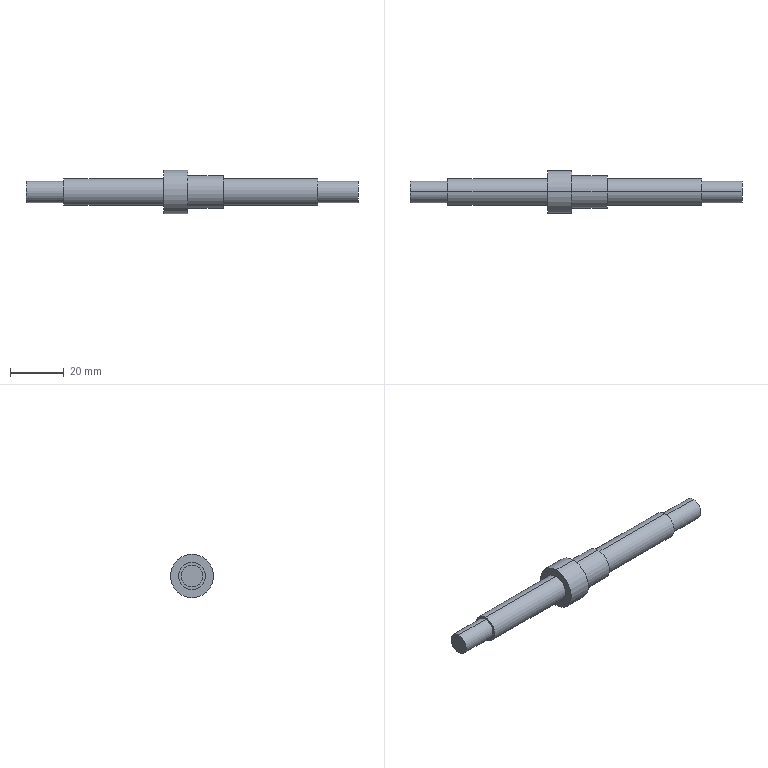Component | SolidWorks | IntermediateAxis-1 | 1 solid | 19 faces | box 123 x 16 x 16 mm | volume 10392 mm3 | cylinder 12 | plane 7 | commonest cylinder face diameters 8 x4 10 x4 12 x2 16 x2 | material AISI 1045 Steel, Cold Drawn
build123d program:
from build123d import *


with BuildPart() as part:
    # Sketch1 → Revolve1 (revolve)
    with BuildSketch(Plane.XY, mode=Mode.PRIVATE) as revolve1_sk:
        Polygon((0, 0), (0, 4), (14, 4), (14, 5), (51, 5), (51, 8), (60, 8), (60, 6), (73, 6), (73, 5), (108, 5), (108, 4), (123, 4), (123, 0), align=None)
    revolve(revolve1_sk.sketch.rotate(Axis((-147.307, 0, 0), (1, 0, 0)), 90), axis=Axis((-147.307, 0, 0), (1, 0, 0)))


solid = part.part

# Placed as in the assembly
solid = solid.moved(Location((116.062, 15.116, 349), (0, 0, 0)))
STEP:
#1=COLOUR_RGB('',0.7922,0.8196,0.9333);
#2=FILL_AREA_STYLE_COLOUR('',#1);
#3=FILL_AREA_STYLE('',(#2));
#4=SURFACE_STYLE_FILL_AREA(#3);
#5=SURFACE_SIDE_STYLE('',(#4));
#6=SURFACE_STYLE_USAGE(.BOTH.,#5);
#7=PRESENTATION_STYLE_ASSIGNMENT((#6));
#8=CARTESIAN_POINT('',(9.412,0.5951,13.898));
#9=VERTEX_POINT('',#8);
#10=CARTESIAN_POINT('',(9.412,0.5951,13.583));
#11=VERTEX_POINT('',#10);
#12=CARTESIAN_POINT('',(9.412,0.5951,13.74));
#13=DIRECTION('',(-1.,0.,0.));
#14=DIRECTION('',(0.,0.,1.));
#15=AXIS2_PLACEMENT_3D('',#12,#13,#14);
#16=CIRCLE('',#15,0.1575);
#17=EDGE_CURVE('',#9,#11,#16,.T.);
#18=ORIENTED_EDGE('',*,*,#17,.T.);
#19=CARTESIAN_POINT('',(8.821,0.5951,13.583));
#20=VERTEX_POINT('',#19);
#21=CARTESIAN_POINT('',(-1.23,0.5951,13.583));
#22=DIRECTION('',(-1.,0.,0.));
#23=VECTOR('',#22,39.37);
#24=LINE('',#21,#23);
#25=EDGE_CURVE('',#11,#20,#24,.T.);
#26=ORIENTED_EDGE('',*,*,#25,.T.);
#27=CARTESIAN_POINT('',(8.821,0.5951,13.898));
#28=VERTEX_POINT('',#27);
#29=CARTESIAN_POINT('',(8.821,0.5951,13.74));
#30=DIRECTION('',(-1.,0.,0.));
#31=DIRECTION('',(0.,0.,1.));
#32=AXIS2_PLACEMENT_3D('',#29,#30,#31);
#33=CIRCLE('',#32,0.1575);
#34=EDGE_CURVE('',#28,#20,#33,.T.);
#35=ORIENTED_EDGE('',*,*,#34,.F.);
#36=CARTESIAN_POINT('',(-1.23,0.5951,13.898));
#37=DIRECTION('',(-1.,0.,0.));
#38=VECTOR('',#37,39.37);
#39=LINE('',#36,#38);
#40=EDGE_CURVE('',#9,#28,#39,.T.);
#41=ORIENTED_EDGE('',*,*,#40,.F.);
#42=EDGE_LOOP('',(#18,#26,#35,#41));
#43=FACE_OUTER_BOUND('',#42,.T.);
#44=CARTESIAN_POINT('',(-1.23,0.5951,13.74));
#45=DIRECTION('',(-1.,0.,0.));
#46=DIRECTION('',(0.,0.,1.));
#47=AXIS2_PLACEMENT_3D('',#44,#45,#46);
#48=CYLINDRICAL_SURFACE('',#47,0.1575);
#49=ADVANCED_FACE('',(#43),#48,.T.);
#50=CARTESIAN_POINT('',(8.821,0.5951,13.937));
#51=VERTEX_POINT('',#50);
#52=CARTESIAN_POINT('',(8.821,0.5951,13.543));
#53=VERTEX_POINT('',#52);
#54=CARTESIAN_POINT('',(8.821,0.5951,13.74));
#55=DIRECTION('',(-1.,0.,0.));
#56=DIRECTION('',(0.,0.,1.));
#57=AXIS2_PLACEMENT_3D('',#54,#55,#56);
#58=CIRCLE('',#57,0.1969);
#59=EDGE_CURVE('',#51,#53,#58,.T.);
#60=ORIENTED_EDGE('',*,*,#59,.T.);
#61=CARTESIAN_POINT('',(7.443,0.5951,13.543));
#62=VERTEX_POINT('',#61);
#63=CARTESIAN_POINT('',(-1.23,0.5951,13.543));
#64=DIRECTION('',(-1.,0.,0.));
#65=VECTOR('',#64,39.37);
#66=LINE('',#63,#65);
#67=EDGE_CURVE('',#53,#62,#66,.T.);
#68=ORIENTED_EDGE('',*,*,#67,.T.);
#69=CARTESIAN_POINT('',(7.443,0.5951,13.937));
#70=VERTEX_POINT('',#69);
#71=CARTESIAN_POINT('',(7.443,0.5951,13.74));
#72=DIRECTION('',(-1.,0.,0.));
#73=DIRECTION('',(0.,0.,1.));
#74=AXIS2_PLACEMENT_3D('',#71,#72,#73);
#75=CIRCLE('',#74,0.1969);
#76=EDGE_CURVE('',#70,#62,#75,.T.);
#77=ORIENTED_EDGE('',*,*,#76,.F.);
#78=CARTESIAN_POINT('',(-1.23,0.5951,13.937));
#79=DIRECTION('',(-1.,0.,0.));
#80=VECTOR('',#79,39.37);
#81=LINE('',#78,#80);
#82=EDGE_CURVE('',#51,#70,#81,.T.);
#83=ORIENTED_EDGE('',*,*,#82,.F.);
#84=EDGE_LOOP('',(#60,#68,#77,#83));
#85=FACE_OUTER_BOUND('',#84,.T.);
#86=CARTESIAN_POINT('',(-1.23,0.5951,13.74));
#87=DIRECTION('',(-1.,0.,0.));
#88=DIRECTION('',(0.,0.,1.));
#89=AXIS2_PLACEMENT_3D('',#86,#87,#88);
#90=CYLINDRICAL_SURFACE('',#89,0.1969);
#91=ADVANCED_FACE('',(#85),#90,.T.);
#92=CARTESIAN_POINT('',(7.443,0.5951,13.976));
#93=VERTEX_POINT('',#92);
#94=CARTESIAN_POINT('',(7.443,0.5951,13.504));
#95=VERTEX_POINT('',#94);
#96=CARTESIAN_POINT('',(7.443,0.5951,13.74));
#97=DIRECTION('',(-1.,0.,0.));
#98=DIRECTION('',(0.,0.,1.));
#99=AXIS2_PLACEMENT_3D('',#96,#97,#98);
#100=CIRCLE('',#99,0.2362);
#101=EDGE_CURVE('',#93,#95,#100,.T.);
#102=ORIENTED_EDGE('',*,*,#101,.T.);
#103=CARTESIAN_POINT('',(6.932,0.5951,13.504));
#104=VERTEX_POINT('',#103);
#105=CARTESIAN_POINT('',(-1.23,0.5951,13.504));
#106=DIRECTION('',(-1.,0.,0.));
#107=VECTOR('',#106,39.37);
#108=LINE('',#105,#107);
#109=EDGE_CURVE('',#95,#104,#108,.T.);
#110=ORIENTED_EDGE('',*,*,#109,.T.);
#111=CARTESIAN_POINT('',(6.932,0.5951,13.976));
#112=VERTEX_POINT('',#111);
#113=CARTESIAN_POINT('',(6.932,0.5951,13.74));
#114=DIRECTION('',(-1.,0.,0.));
#115=DIRECTION('',(0.,0.,1.));
#116=AXIS2_PLACEMENT_3D('',#113,#114,#115);
#117=CIRCLE('',#116,0.2362);
#118=EDGE_CURVE('',#112,#104,#117,.T.);
#119=ORIENTED_EDGE('',*,*,#118,.F.);
#120=CARTESIAN_POINT('',(-1.23,0.5951,13.976));
#121=DIRECTION('',(-1.,0.,0.));
#122=VECTOR('',#121,39.37);
#123=LINE('',#120,#122);
#124=EDGE_CURVE('',#93,#112,#123,.T.);
#125=ORIENTED_EDGE('',*,*,#124,.F.);
#126=EDGE_LOOP('',(#102,#110,#119,#125));
#127=FACE_OUTER_BOUND('',#126,.T.);
#128=CARTESIAN_POINT('',(-1.23,0.5951,13.74));
#129=DIRECTION('',(-1.,0.,0.));
#130=DIRECTION('',(0.,0.,1.));
#131=AXIS2_PLACEMENT_3D('',#128,#129,#130);
#132=CYLINDRICAL_SURFACE('',#131,0.2362);
#133=ADVANCED_FACE('',(#127),#132,.T.);
#134=CARTESIAN_POINT('',(6.932,0.5951,14.055));
#135=VERTEX_POINT('',#134);
#136=CARTESIAN_POINT('',(6.932,0.5951,13.425));
#137=VERTEX_POINT('',#136);
#138=CARTESIAN_POINT('',(6.932,0.5951,13.74));
#139=DIRECTION('',(-1.,0.,0.));
#140=DIRECTION('',(0.,0.,1.));
#141=AXIS2_PLACEMENT_3D('',#138,#139,#140);
#142=CIRCLE('',#141,0.315);
#143=EDGE_CURVE('',#135,#137,#142,.T.);
#144=ORIENTED_EDGE('',*,*,#143,.T.);
#145=CARTESIAN_POINT('',(6.577,0.5951,13.425));
#146=VERTEX_POINT('',#145);
#147=CARTESIAN_POINT('',(-1.23,0.5951,13.425));
#148=DIRECTION('',(-1.,0.,0.));
#149=VECTOR('',#148,39.37);
#150=LINE('',#147,#149);
#151=EDGE_CURVE('',#137,#146,#150,.T.);
#152=ORIENTED_EDGE('',*,*,#151,.T.);
#153=CARTESIAN_POINT('',(6.577,0.5951,14.055));
#154=VERTEX_POINT('',#153);
#155=CARTESIAN_POINT('',(6.577,0.5951,13.74));
#156=DIRECTION('',(-1.,0.,0.));
#157=DIRECTION('',(0.,0.,1.));
#158=AXIS2_PLACEMENT_3D('',#155,#156,#157);
#159=CIRCLE('',#158,0.315);
#160=EDGE_CURVE('',#154,#146,#159,.T.);
#161=ORIENTED_EDGE('',*,*,#160,.F.);
#162=CARTESIAN_POINT('',(-1.23,0.5951,14.055));
#163=DIRECTION('',(-1.,0.,0.));
#164=VECTOR('',#163,39.37);
#165=LINE('',#162,#164);
#166=EDGE_CURVE('',#135,#154,#165,.T.);
#167=ORIENTED_EDGE('',*,*,#166,.F.);
#168=EDGE_LOOP('',(#144,#152,#161,#167));
#169=FACE_OUTER_BOUND('',#168,.T.);
#170=CARTESIAN_POINT('',(-1.23,0.5951,13.74));
#171=DIRECTION('',(-1.,0.,0.));
#172=DIRECTION('',(0.,0.,1.));
#173=AXIS2_PLACEMENT_3D('',#170,#171,#172);
#174=CYLINDRICAL_SURFACE('',#173,0.315);
#175=ADVANCED_FACE('',(#169),#174,.T.);
#176=CARTESIAN_POINT('',(6.577,0.5951,13.937));
#177=VERTEX_POINT('',#176);
#178=CARTESIAN_POINT('',(6.577,0.5951,13.543));
#179=VERTEX_POINT('',#178);
#180=CARTESIAN_POINT('',(6.577,0.5951,13.74));
#181=DIRECTION('',(-1.,0.,0.));
#182=DIRECTION('',(0.,0.,1.));
#183=AXIS2_PLACEMENT_3D('',#180,#181,#182);
#184=CIRCLE('',#183,0.1969);
#185=EDGE_CURVE('',#177,#179,#184,.T.);
#186=ORIENTED_EDGE('',*,*,#185,.T.);
#187=CARTESIAN_POINT('',(5.121,0.5951,13.543));
#188=VERTEX_POINT('',#187);
#189=CARTESIAN_POINT('',(-1.23,0.5951,13.543));
#190=DIRECTION('',(-1.,0.,0.));
#191=VECTOR('',#190,39.37);
#192=LINE('',#189,#191);
#193=EDGE_CURVE('',#179,#188,#192,.T.);
#194=ORIENTED_EDGE('',*,*,#193,.T.);
#195=CARTESIAN_POINT('',(5.121,0.5951,13.937));
#196=VERTEX_POINT('',#195);
#197=CARTESIAN_POINT('',(5.121,0.5951,13.74));
#198=DIRECTION('',(-1.,0.,0.));
#199=DIRECTION('',(0.,0.,1.));
#200=AXIS2_PLACEMENT_3D('',#197,#198,#199);
#201=CIRCLE('',#200,0.1969);
#202=EDGE_CURVE('',#196,#188,#201,.T.);
#203=ORIENTED_EDGE('',*,*,#202,.F.);
#204=CARTESIAN_POINT('',(-1.23,0.5951,13.937));
#205=DIRECTION('',(-1.,0.,0.));
#206=VECTOR('',#205,39.37);
#207=LINE('',#204,#206);
#208=EDGE_CURVE('',#177,#196,#207,.T.);
#209=ORIENTED_EDGE('',*,*,#208,.F.);
#210=EDGE_LOOP('',(#186,#194,#203,#209));
#211=FACE_OUTER_BOUND('',#210,.T.);
#212=CARTESIAN_POINT('',(-1.23,0.5951,13.74));
#213=DIRECTION('',(-1.,0.,0.));
#214=DIRECTION('',(0.,0.,1.));
#215=AXIS2_PLACEMENT_3D('',#212,#213,#214);
#216=CYLINDRICAL_SURFACE('',#215,0.1969);
#217=ADVANCED_FACE('',(#211),#216,.T.);
#218=CARTESIAN_POINT('',(5.121,0.5951,13.898));
#219=VERTEX_POINT('',#218);
#220=CARTESIAN_POINT('',(5.121,0.5951,13.583));
#221=VERTEX_POINT('',#220);
#222=CARTESIAN_POINT('',(5.121,0.5951,13.74));
#223=DIRECTION('',(-1.,0.,0.));
#224=DIRECTION('',(0.,0.,1.));
#225=AXIS2_PLACEMENT_3D('',#222,#223,#224);
#226=CIRCLE('',#225,0.1575);
#227=EDGE_CURVE('',#219,#221,#226,.T.);
#228=ORIENTED_EDGE('',*,*,#227,.T.);
#229=CARTESIAN_POINT('',(4.569,0.5951,13.583));
#230=VERTEX_POINT('',#229);
#231=CARTESIAN_POINT('',(-1.23,0.5951,13.583));
#232=DIRECTION('',(-1.,0.,0.));
#233=VECTOR('',#232,39.37);
#234=LINE('',#231,#233);
#235=EDGE_CURVE('',#221,#230,#234,.T.);
#236=ORIENTED_EDGE('',*,*,#235,.T.);
#237=CARTESIAN_POINT('',(4.569,0.5951,13.898));
#238=VERTEX_POINT('',#237);
#239=CARTESIAN_POINT('',(4.569,0.5951,13.74));
#240=DIRECTION('',(-1.,0.,0.));
#241=DIRECTION('',(0.,0.,1.));
#242=AXIS2_PLACEMENT_3D('',#239,#240,#241);
#243=CIRCLE('',#242,0.1575);
#244=EDGE_CURVE('',#238,#230,#243,.T.);
#245=ORIENTED_EDGE('',*,*,#244,.F.);
#246=CARTESIAN_POINT('',(-1.23,0.5951,13.898));
#247=DIRECTION('',(-1.,0.,0.));
#248=VECTOR('',#247,39.37);
#249=LINE('',#246,#248);
#250=EDGE_CURVE('',#219,#238,#249,.T.);
#251=ORIENTED_EDGE('',*,*,#250,.F.);
#252=EDGE_LOOP('',(#228,#236,#245,#251));
#253=FACE_OUTER_BOUND('',#252,.T.);
#254=CARTESIAN_POINT('',(-1.23,0.5951,13.74));
#255=DIRECTION('',(-1.,0.,0.));
#256=DIRECTION('',(0.,0.,1.));
#257=AXIS2_PLACEMENT_3D('',#254,#255,#256);
#258=CYLINDRICAL_SURFACE('',#257,0.1575);
#259=ADVANCED_FACE('',(#253),#258,.T.);
#260=ORIENTED_EDGE('',*,*,#244,.T.);
#261=CARTESIAN_POINT('',(4.569,0.5951,13.74));
#262=DIRECTION('',(-1.,0.,0.));
#263=DIRECTION('',(0.,0.,1.));
#264=AXIS2_PLACEMENT_3D('',#261,#262,#263);
#265=CIRCLE('',#264,0.1575);
#266=EDGE_CURVE('',#230,#238,#265,.T.);
#267=ORIENTED_EDGE('',*,*,#266,.T.);
#268=EDGE_LOOP('',(#260,#267));
#269=FACE_OUTER_BOUND('',#268,.T.);
#270=CARTESIAN_POINT('',(4.569,0.5951,13.74));
#271=DIRECTION('',(1.,0.,0.));
#272=DIRECTION('',(0.,0.,-1.));
#273=AXIS2_PLACEMENT_3D('',#270,#271,#272);
#274=PLANE('',#273);
#275=ADVANCED_FACE('',(#269),#274,.F.);
#276=ORIENTED_EDGE('',*,*,#235,.F.);
#277=CARTESIAN_POINT('',(5.121,0.5951,13.74));
#278=DIRECTION('',(-1.,0.,0.));
#279=DIRECTION('',(0.,0.,1.));
#280=AXIS2_PLACEMENT_3D('',#277,#278,#279);
#281=CIRCLE('',#280,0.1575);
#282=EDGE_CURVE('',#221,#219,#281,.T.);
#283=ORIENTED_EDGE('',*,*,#282,.T.);
#284=ORIENTED_EDGE('',*,*,#250,.T.);
#285=ORIENTED_EDGE('',*,*,#266,.F.);
#286=EDGE_LOOP('',(#276,#283,#284,#285));
#287=FACE_OUTER_BOUND('',#286,.T.);
#288=CARTESIAN_POINT('',(-1.23,0.5951,13.74));
#289=DIRECTION('',(-1.,0.,0.));
#290=DIRECTION('',(0.,0.,1.));
#291=AXIS2_PLACEMENT_3D('',#288,#289,#290);
#292=CYLINDRICAL_SURFACE('',#291,0.1575);
#293=ADVANCED_FACE('',(#287),#292,.T.);
#294=ORIENTED_EDGE('',*,*,#227,.F.);
#295=ORIENTED_EDGE('',*,*,#282,.F.);
#296=EDGE_LOOP('',(#294,#295));
#297=FACE_BOUND('',#296,.T.);
#298=ORIENTED_EDGE('',*,*,#202,.T.);
#299=CARTESIAN_POINT('',(5.121,0.5951,13.74));
#300=DIRECTION('',(-1.,0.,0.));
#301=DIRECTION('',(0.,0.,1.));
#302=AXIS2_PLACEMENT_3D('',#299,#300,#301);
#303=CIRCLE('',#302,0.1969);
#304=EDGE_CURVE('',#188,#196,#303,.T.);
#305=ORIENTED_EDGE('',*,*,#304,.T.);
#306=EDGE_LOOP('',(#298,#305));
#307=FACE_OUTER_BOUND('',#306,.T.);
#308=CARTESIAN_POINT('',(5.121,0.7526,13.74));
#309=DIRECTION('',(1.,0.,0.));
#310=DIRECTION('',(0.,0.,-1.));
#311=AXIS2_PLACEMENT_3D('',#308,#309,#310);
#312=PLANE('',#311);
#313=ADVANCED_FACE('',(#297,#307),#312,.F.);
#314=ORIENTED_EDGE('',*,*,#193,.F.);
#315=CARTESIAN_POINT('',(6.577,0.5951,13.74));
#316=DIRECTION('',(-1.,0.,0.));
#317=DIRECTION('',(0.,0.,1.));
#318=AXIS2_PLACEMENT_3D('',#315,#316,#317);
#319=CIRCLE('',#318,0.1969);
#320=EDGE_CURVE('',#179,#177,#319,.T.);
#321=ORIENTED_EDGE('',*,*,#320,.T.);
#322=ORIENTED_EDGE('',*,*,#208,.T.);
#323=ORIENTED_EDGE('',*,*,#304,.F.);
#324=EDGE_LOOP('',(#314,#321,#322,#323));
#325=FACE_OUTER_BOUND('',#324,.T.);
#326=CARTESIAN_POINT('',(-1.23,0.5951,13.74));
#327=DIRECTION('',(-1.,0.,0.));
#328=DIRECTION('',(0.,0.,1.));
#329=AXIS2_PLACEMENT_3D('',#326,#327,#328);
#330=CYLINDRICAL_SURFACE('',#329,0.1969);
#331=ADVANCED_FACE('',(#325),#330,.T.);
#332=ORIENTED_EDGE('',*,*,#185,.F.);
#333=ORIENTED_EDGE('',*,*,#320,.F.);
#334=EDGE_LOOP('',(#332,#333));
#335=FACE_BOUND('',#334,.T.);
#336=ORIENTED_EDGE('',*,*,#160,.T.);
#337=CARTESIAN_POINT('',(6.577,0.5951,13.74));
#338=DIRECTION('',(-1.,0.,0.));
#339=DIRECTION('',(0.,0.,1.));
#340=AXIS2_PLACEMENT_3D('',#337,#338,#339);
#341=CIRCLE('',#340,0.315);
#342=EDGE_CURVE('',#146,#154,#341,.T.);
#343=ORIENTED_EDGE('',*,*,#342,.T.);
#344=EDGE_LOOP('',(#336,#343));
#345=FACE_OUTER_BOUND('',#344,.T.);
#346=CARTESIAN_POINT('',(6.577,0.792,13.74));
#347=DIRECTION('',(1.,0.,0.));
#348=DIRECTION('',(0.,0.,-1.));
#349=AXIS2_PLACEMENT_3D('',#346,#347,#348);
#350=PLANE('',#349);
#351=ADVANCED_FACE('',(#335,#345),#350,.F.);
#352=ORIENTED_EDGE('',*,*,#151,.F.);
#353=CARTESIAN_POINT('',(6.932,0.5951,13.74));
#354=DIRECTION('',(-1.,0.,0.));
#355=DIRECTION('',(0.,0.,1.));
#356=AXIS2_PLACEMENT_3D('',#353,#354,#355);
#357=CIRCLE('',#356,0.315);
#358=EDGE_CURVE('',#137,#135,#357,.T.);
#359=ORIENTED_EDGE('',*,*,#358,.T.);
#360=ORIENTED_EDGE('',*,*,#166,.T.);
#361=ORIENTED_EDGE('',*,*,#342,.F.);
#362=EDGE_LOOP('',(#352,#359,#360,#361));
#363=FACE_OUTER_BOUND('',#362,.T.);
#364=CARTESIAN_POINT('',(-1.23,0.5951,13.74));
#365=DIRECTION('',(-1.,0.,0.));
#366=DIRECTION('',(0.,0.,1.));
#367=AXIS2_PLACEMENT_3D('',#364,#365,#366);
#368=CYLINDRICAL_SURFACE('',#367,0.315);
#369=ADVANCED_FACE('',(#363),#368,.T.);
#370=ORIENTED_EDGE('',*,*,#143,.F.);
#371=ORIENTED_EDGE('',*,*,#358,.F.);
#372=EDGE_LOOP('',(#370,#371));
#373=FACE_OUTER_BOUND('',#372,.T.);
#374=ORIENTED_EDGE('',*,*,#118,.T.);
#375=CARTESIAN_POINT('',(6.932,0.5951,13.74));
#376=DIRECTION('',(-1.,0.,0.));
#377=DIRECTION('',(0.,0.,1.));
#378=AXIS2_PLACEMENT_3D('',#375,#376,#377);
#379=CIRCLE('',#378,0.2362);
#380=EDGE_CURVE('',#104,#112,#379,.T.);
#381=ORIENTED_EDGE('',*,*,#380,.T.);
#382=EDGE_LOOP('',(#374,#381));
#383=FACE_BOUND('',#382,.T.);
#384=CARTESIAN_POINT('',(6.932,0.9101,13.74));
#385=DIRECTION('',(-1.,0.,0.));
#386=DIRECTION('',(0.,0.,1.));
#387=AXIS2_PLACEMENT_3D('',#384,#385,#386);
#388=PLANE('',#387);
#389=ADVANCED_FACE('',(#373,#383),#388,.F.);
#390=ORIENTED_EDGE('',*,*,#109,.F.);
#391=CARTESIAN_POINT('',(7.443,0.5951,13.74));
#392=DIRECTION('',(-1.,0.,0.));
#393=DIRECTION('',(0.,0.,1.));
#394=AXIS2_PLACEMENT_3D('',#391,#392,#393);
#395=CIRCLE('',#394,0.2362);
#396=EDGE_CURVE('',#95,#93,#395,.T.);
#397=ORIENTED_EDGE('',*,*,#396,.T.);
#398=ORIENTED_EDGE('',*,*,#124,.T.);
#399=ORIENTED_EDGE('',*,*,#380,.F.);
#400=EDGE_LOOP('',(#390,#397,#398,#399));
#401=FACE_OUTER_BOUND('',#400,.T.);
#402=CARTESIAN_POINT('',(-1.23,0.5951,13.74));
#403=DIRECTION('',(-1.,0.,0.));
#404=DIRECTION('',(0.,0.,1.));
#405=AXIS2_PLACEMENT_3D('',#402,#403,#404);
#406=CYLINDRICAL_SURFACE('',#405,0.2362);
#407=ADVANCED_FACE('',(#401),#406,.T.);
#408=ORIENTED_EDGE('',*,*,#101,.F.);
#409=ORIENTED_EDGE('',*,*,#396,.F.);
#410=EDGE_LOOP('',(#408,#409));
#411=FACE_OUTER_BOUND('',#410,.T.);
#412=ORIENTED_EDGE('',*,*,#76,.T.);
#413=CARTESIAN_POINT('',(7.443,0.5951,13.74));
#414=DIRECTION('',(-1.,0.,0.));
#415=DIRECTION('',(0.,0.,1.));
#416=AXIS2_PLACEMENT_3D('',#413,#414,#415);
#417=CIRCLE('',#416,0.1969);
#418=EDGE_CURVE('',#62,#70,#417,.T.);
#419=ORIENTED_EDGE('',*,*,#418,.T.);
#420=EDGE_LOOP('',(#412,#419));
#421=FACE_BOUND('',#420,.T.);
#422=CARTESIAN_POINT('',(7.443,0.8313,13.74));
#423=DIRECTION('',(-1.,0.,0.));
#424=DIRECTION('',(0.,0.,1.));
#425=AXIS2_PLACEMENT_3D('',#422,#423,#424);
#426=PLANE('',#425);
#427=ADVANCED_FACE('',(#411,#421),#426,.F.);
#428=ORIENTED_EDGE('',*,*,#67,.F.);
#429=CARTESIAN_POINT('',(8.821,0.5951,13.74));
#430=DIRECTION('',(-1.,0.,0.));
#431=DIRECTION('',(0.,0.,1.));
#432=AXIS2_PLACEMENT_3D('',#429,#430,#431);
#433=CIRCLE('',#432,0.1969);
#434=EDGE_CURVE('',#53,#51,#433,.T.);
#435=ORIENTED_EDGE('',*,*,#434,.T.);
#436=ORIENTED_EDGE('',*,*,#82,.T.);
#437=ORIENTED_EDGE('',*,*,#418,.F.);
#438=EDGE_LOOP('',(#428,#435,#436,#437));
#439=FACE_OUTER_BOUND('',#438,.T.);
#440=CARTESIAN_POINT('',(-1.23,0.5951,13.74));
#441=DIRECTION('',(-1.,0.,0.));
#442=DIRECTION('',(0.,0.,1.));
#443=AXIS2_PLACEMENT_3D('',#440,#441,#442);
#444=CYLINDRICAL_SURFACE('',#443,0.1969);
#445=ADVANCED_FACE('',(#439),#444,.T.);
#446=ORIENTED_EDGE('',*,*,#59,.F.);
#447=ORIENTED_EDGE('',*,*,#434,.F.);
#448=EDGE_LOOP('',(#446,#447));
#449=FACE_OUTER_BOUND('',#448,.T.);
#450=ORIENTED_EDGE('',*,*,#34,.T.);
#451=CARTESIAN_POINT('',(8.821,0.5951,13.74));
#452=DIRECTION('',(-1.,0.,0.));
#453=DIRECTION('',(0.,0.,1.));
#454=AXIS2_PLACEMENT_3D('',#451,#452,#453);
#455=CIRCLE('',#454,0.1575);
#456=EDGE_CURVE('',#20,#28,#455,.T.);
#457=ORIENTED_EDGE('',*,*,#456,.T.);
#458=EDGE_LOOP('',(#450,#457));
#459=FACE_BOUND('',#458,.T.);
#460=CARTESIAN_POINT('',(8.821,0.792,13.74));
#461=DIRECTION('',(-1.,0.,0.));
#462=DIRECTION('',(0.,0.,1.));
#463=AXIS2_PLACEMENT_3D('',#460,#461,#462);
#464=PLANE('',#463);
#465=ADVANCED_FACE('',(#449,#459),#464,.F.);
#466=ORIENTED_EDGE('',*,*,#25,.F.);
#467=CARTESIAN_POINT('',(9.412,0.5951,13.74));
#468=DIRECTION('',(-1.,0.,0.));
#469=DIRECTION('',(0.,0.,1.));
#470=AXIS2_PLACEMENT_3D('',#467,#468,#469);
#471=CIRCLE('',#470,0.1575);
#472=EDGE_CURVE('',#11,#9,#471,.T.);
#473=ORIENTED_EDGE('',*,*,#472,.T.);
#474=ORIENTED_EDGE('',*,*,#40,.T.);
#475=ORIENTED_EDGE('',*,*,#456,.F.);
#476=EDGE_LOOP('',(#466,#473,#474,#475));
#477=FACE_OUTER_BOUND('',#476,.T.);
#478=CARTESIAN_POINT('',(-1.23,0.5951,13.74));
#479=DIRECTION('',(-1.,0.,0.));
#480=DIRECTION('',(0.,0.,1.));
#481=AXIS2_PLACEMENT_3D('',#478,#479,#480);
#482=CYLINDRICAL_SURFACE('',#481,0.1575);
#483=ADVANCED_FACE('',(#477),#482,.T.);
#484=ORIENTED_EDGE('',*,*,#17,.F.);
#485=ORIENTED_EDGE('',*,*,#472,.F.);
#486=EDGE_LOOP('',(#484,#485));
#487=FACE_OUTER_BOUND('',#486,.T.);
#488=CARTESIAN_POINT('',(9.412,0.7526,13.74));
#489=DIRECTION('',(-1.,0.,0.));
#490=DIRECTION('',(0.,0.,1.));
#491=AXIS2_PLACEMENT_3D('',#488,#489,#490);
#492=PLANE('',#491);
#493=ADVANCED_FACE('',(#487),#492,.F.);
#494=CLOSED_SHELL('',(#49,#91,#133,#175,#217,#259,#275,#293,#313,#331,#351,#369,#389,#407,#427,#445,#465,#483,#493));
#495=MANIFOLD_SOLID_BREP('',#494);
#496=STYLED_ITEM('',(#7),#495);
#497=(LENGTH_UNIT()NAMED_UNIT(*)SI_UNIT($,.METRE.));
#498=LENGTH_MEASURE_WITH_UNIT(LENGTH_MEASURE(0.0254),#497);
#499=DIMENSIONAL_EXPONENTS(1.,0.,0.,0.,0.,0.,0.);
#500=(CONVERSION_BASED_UNIT('',#498)LENGTH_UNIT()NAMED_UNIT(#499));
#501=UNCERTAINTY_MEASURE_WITH_UNIT(LENGTH_MEASURE(0.00001),#500,'','');
#502=(NAMED_UNIT(*)PLANE_ANGLE_UNIT()SI_UNIT($,.RADIAN.));
#503=(NAMED_UNIT(*)SI_UNIT($,.STERADIAN.)SOLID_ANGLE_UNIT());
#504=(GEOMETRIC_REPRESENTATION_CONTEXT(3)GLOBAL_UNCERTAINTY_ASSIGNED_CONTEXT((#501))GLOBAL_UNIT_ASSIGNED_CONTEXT((#500,#502,#503))REPRESENTATION_CONTEXT('',''));
#505=MECHANICAL_DESIGN_GEOMETRIC_PRESENTATION_REPRESENTATION('',(#496),#504);
#506=CARTESIAN_POINT('',(0.,0.,0.));
#507=DIRECTION('',(0.,0.,1.));
#508=DIRECTION('',(1.,0.,0.));
#509=AXIS2_PLACEMENT_3D('',#506,#507,#508);
#510=(LENGTH_UNIT()NAMED_UNIT(*)SI_UNIT($,.METRE.));
#511=LENGTH_MEASURE_WITH_UNIT(LENGTH_MEASURE(0.0254),#510);
#512=DIMENSIONAL_EXPONENTS(1.,0.,0.,0.,0.,0.,0.);
#513=(CONVERSION_BASED_UNIT('',#511)LENGTH_UNIT()NAMED_UNIT(#512));
#514=UNCERTAINTY_MEASURE_WITH_UNIT(LENGTH_MEASURE(0.00001),#513,'','');
#515=(NAMED_UNIT(*)PLANE_ANGLE_UNIT()SI_UNIT($,.RADIAN.));
#516=(NAMED_UNIT(*)SI_UNIT($,.STERADIAN.)SOLID_ANGLE_UNIT());
#517=(GEOMETRIC_REPRESENTATION_CONTEXT(3)GLOBAL_UNCERTAINTY_ASSIGNED_CONTEXT((#514))GLOBAL_UNIT_ASSIGNED_CONTEXT((#513,#515,#516))REPRESENTATION_CONTEXT('',''));
#518=ADVANCED_BREP_SHAPE_REPRESENTATION('',(#495,#509),#517);
#519=PRESENTATION_LAYER_ASSIGNMENT('','',(#496));